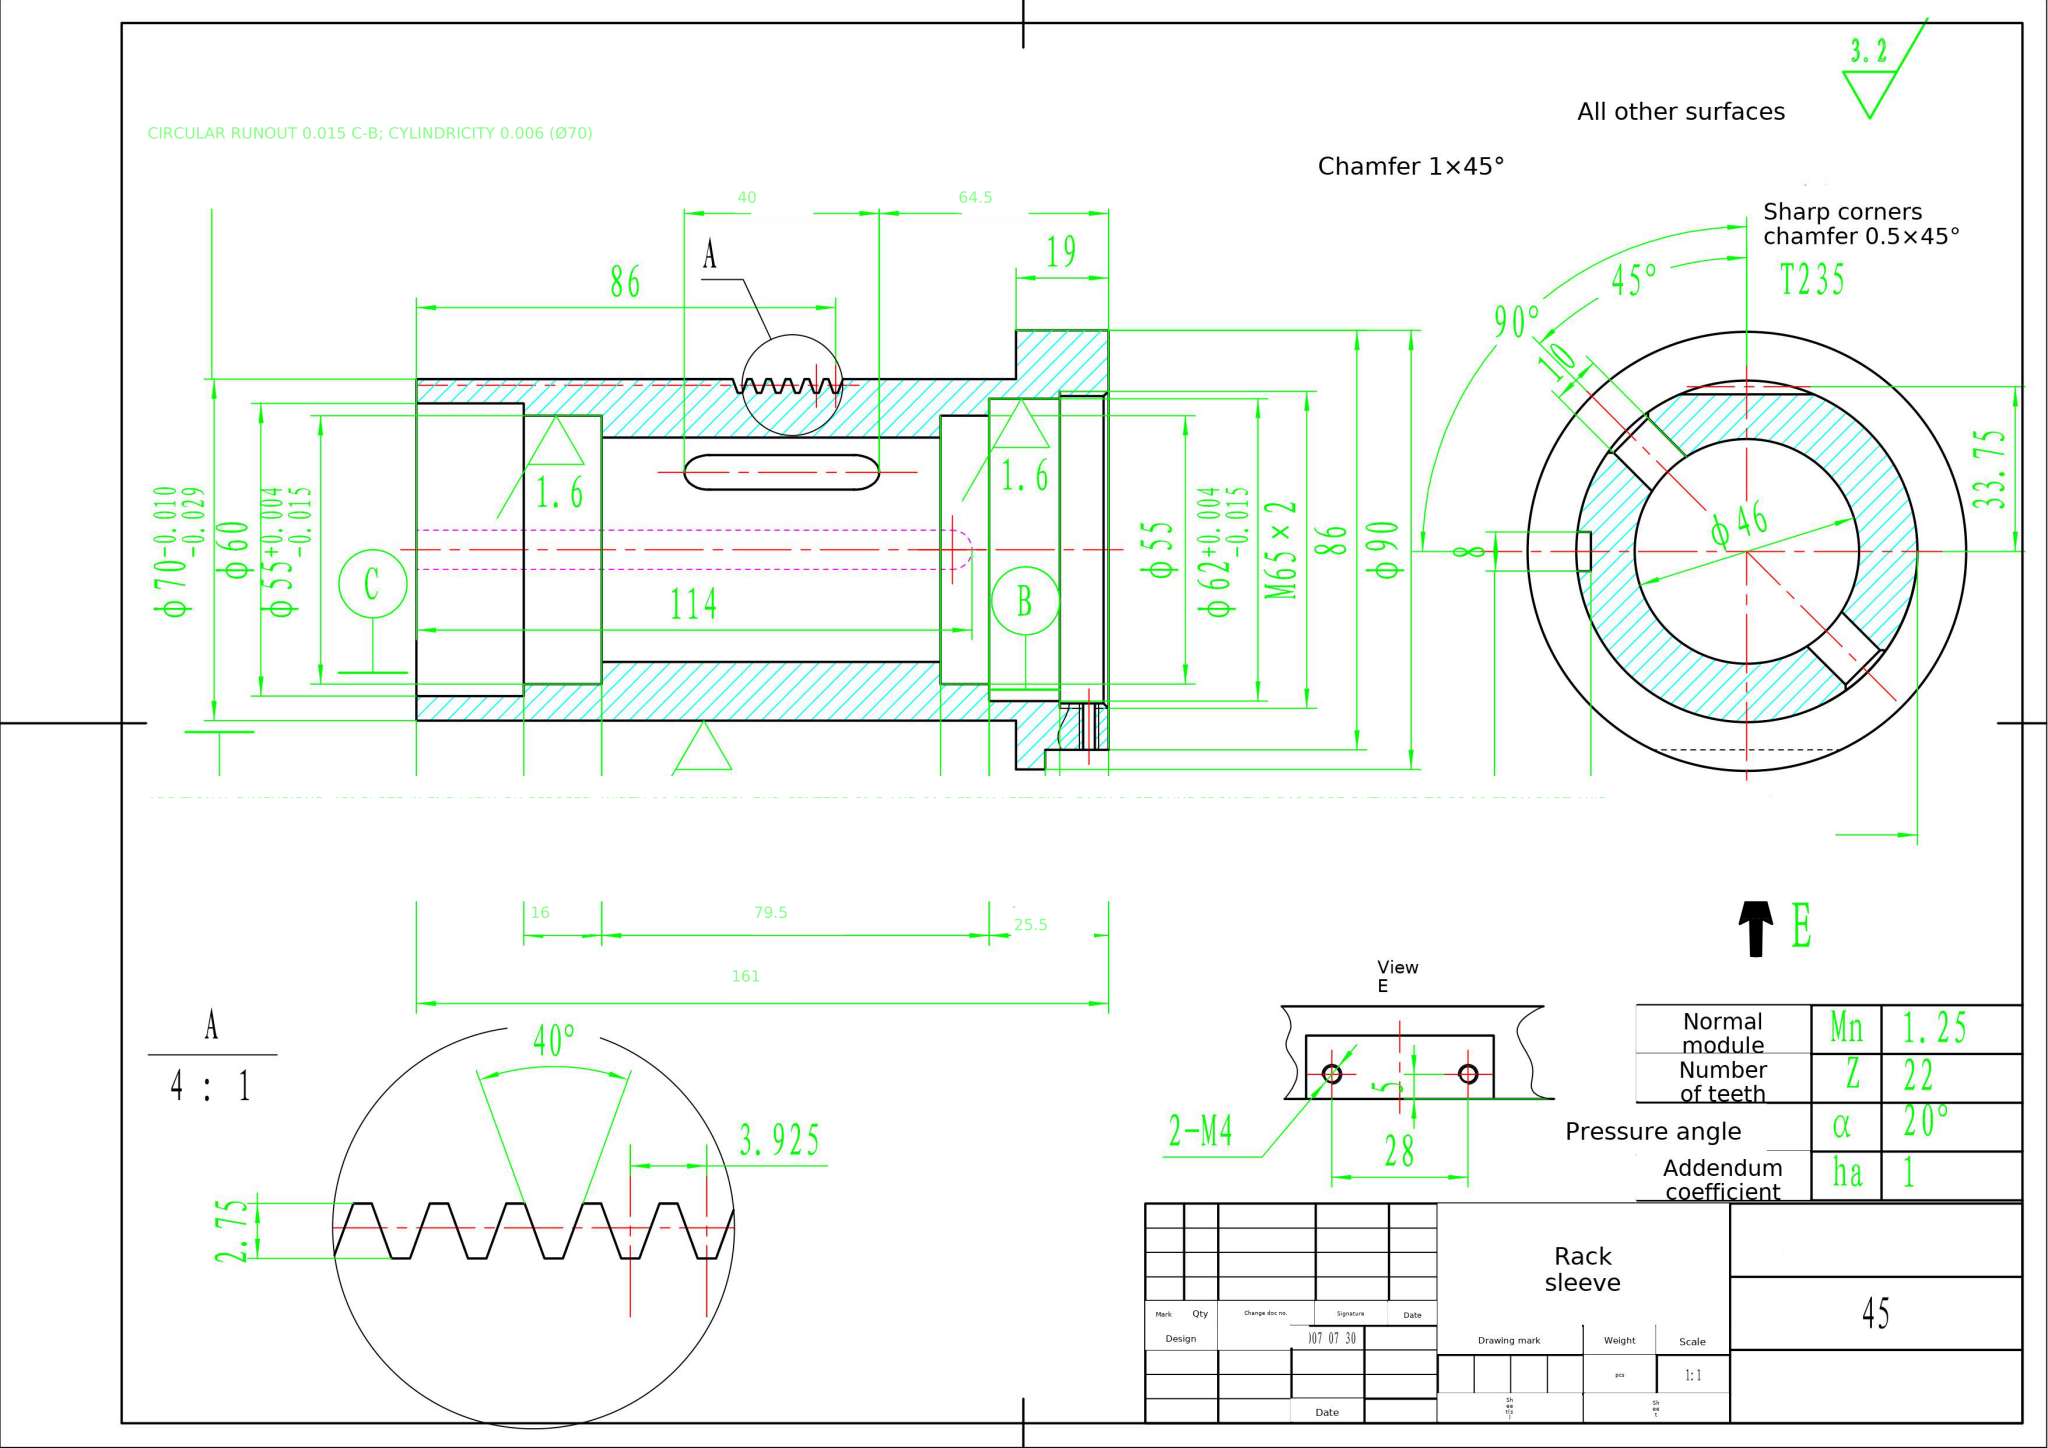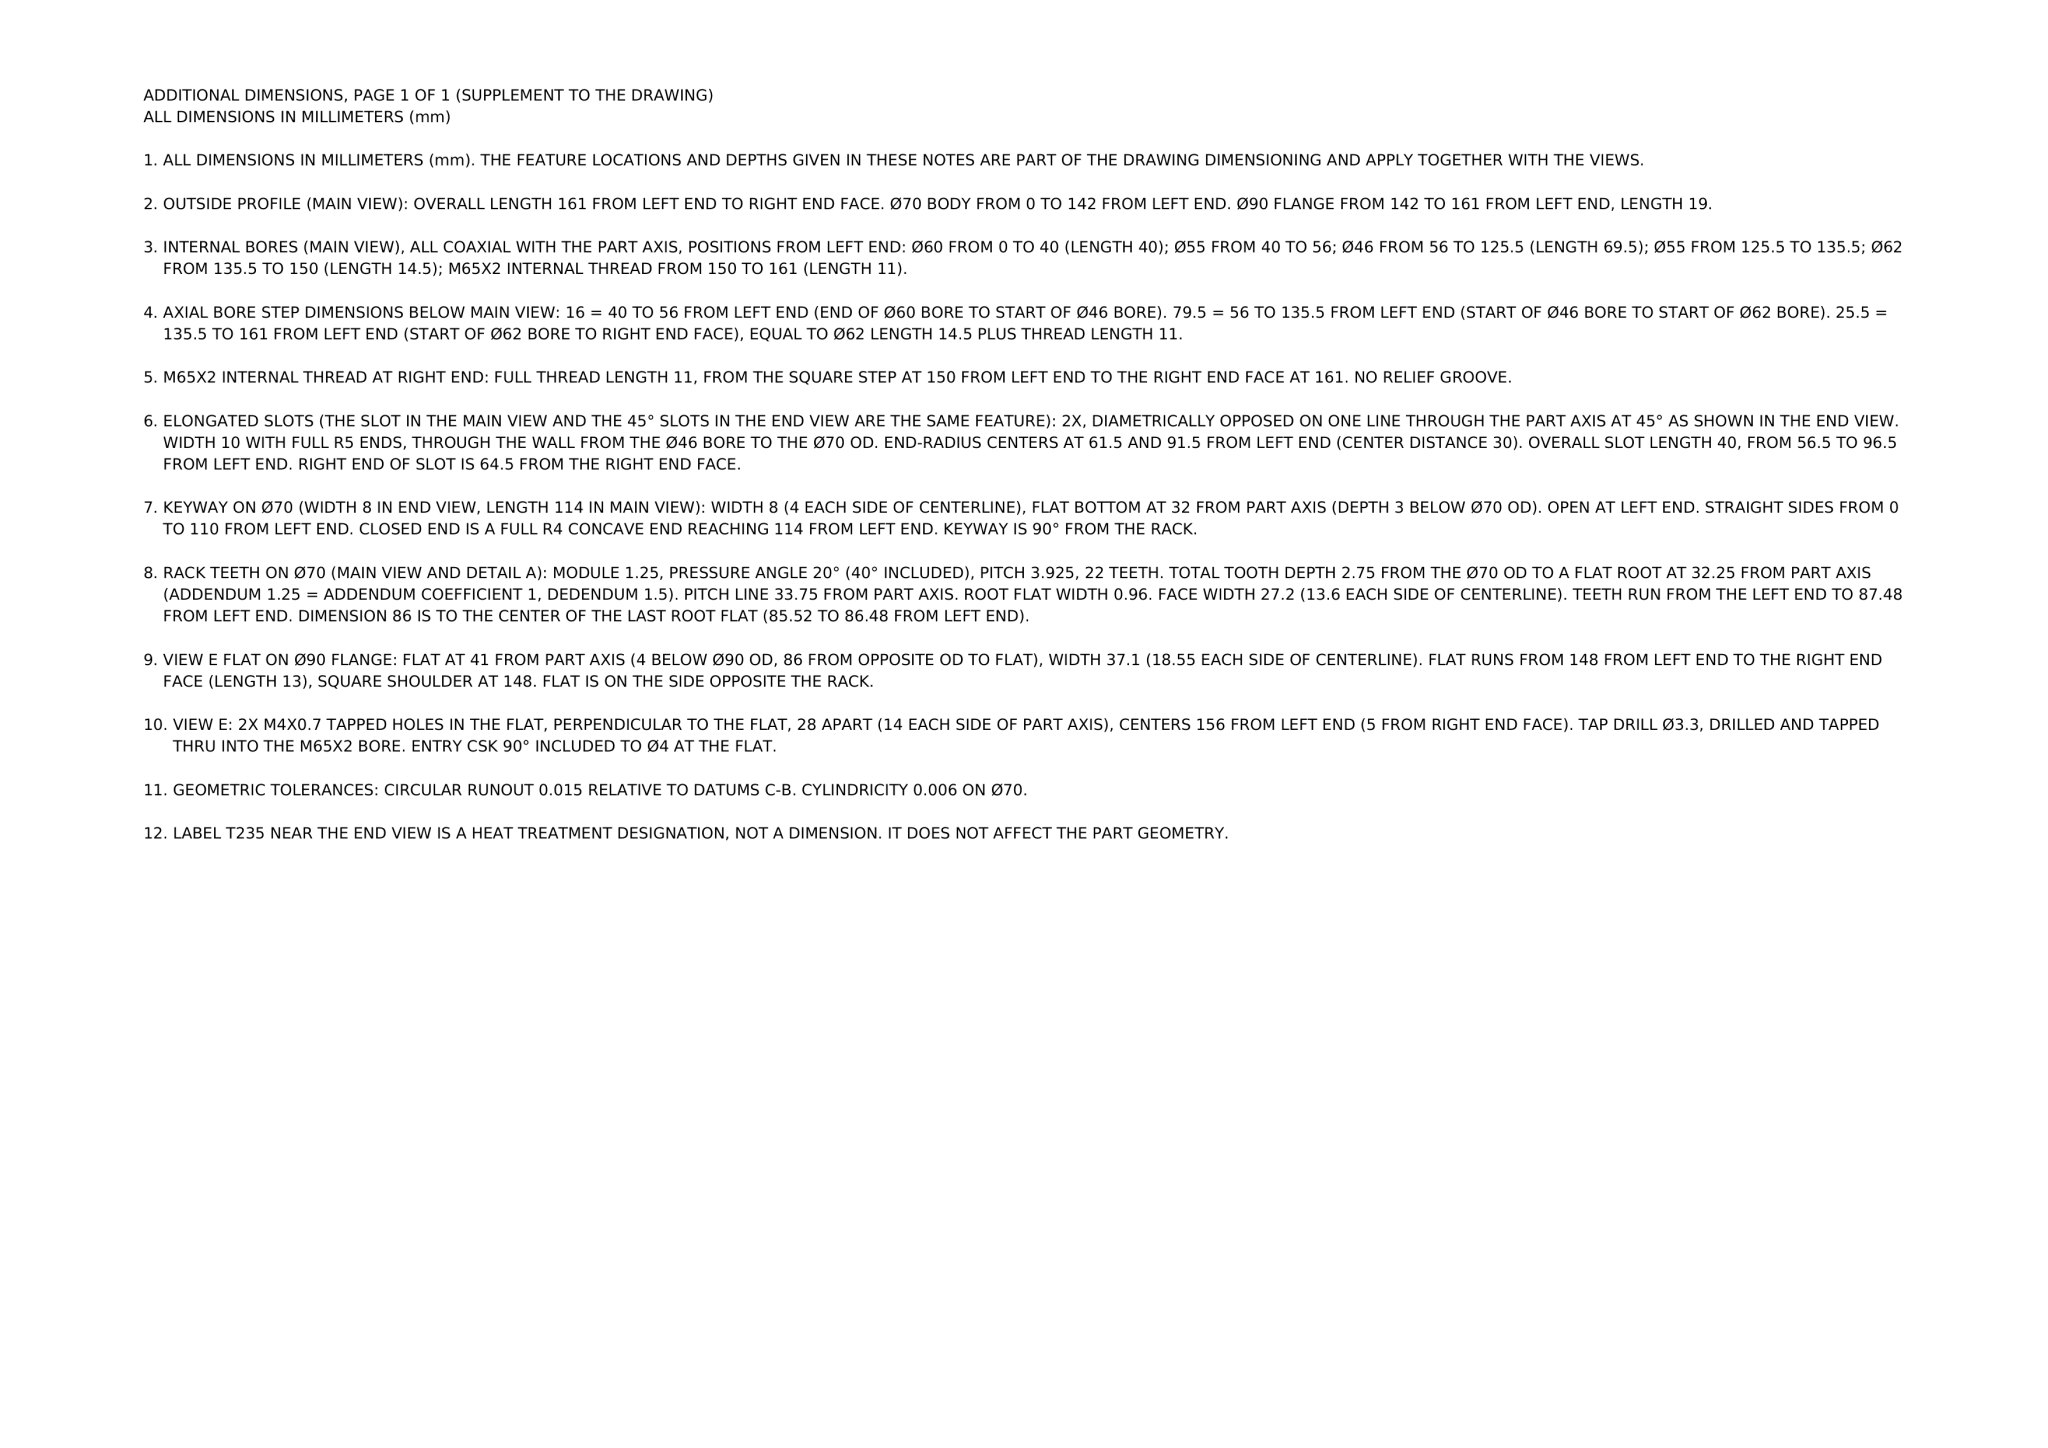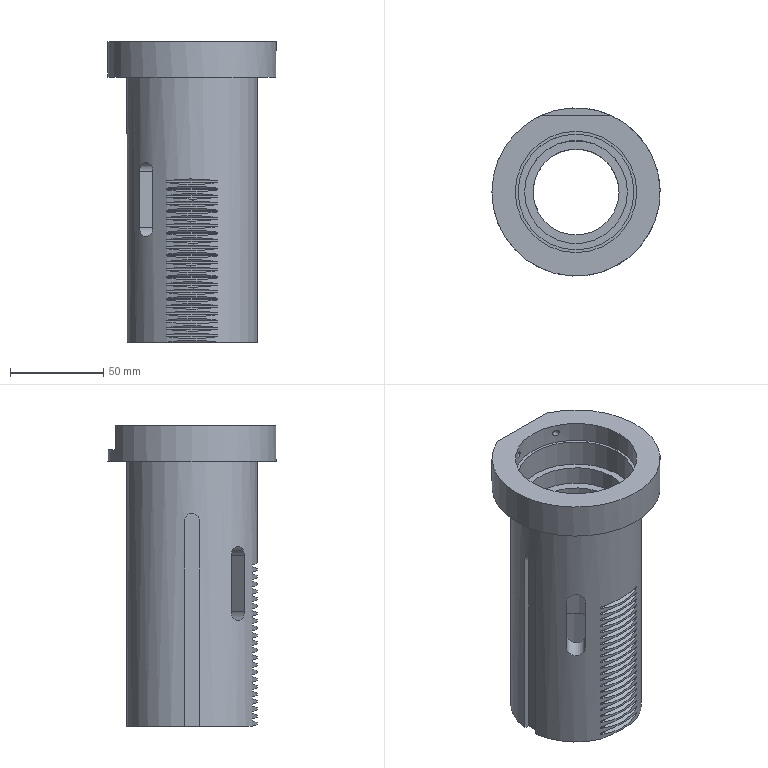Part | NX | mm | 1 solid | 102 faces | box 90 x 90 x 161 mm | volume 281449 mm3 | plane 85 | cylinder 15 | cone 2 | commonest cylinder face diameters 10 x4 55 x2 3.3 x2 70 x1 46 x1 60 x1 90 x1 65 x1